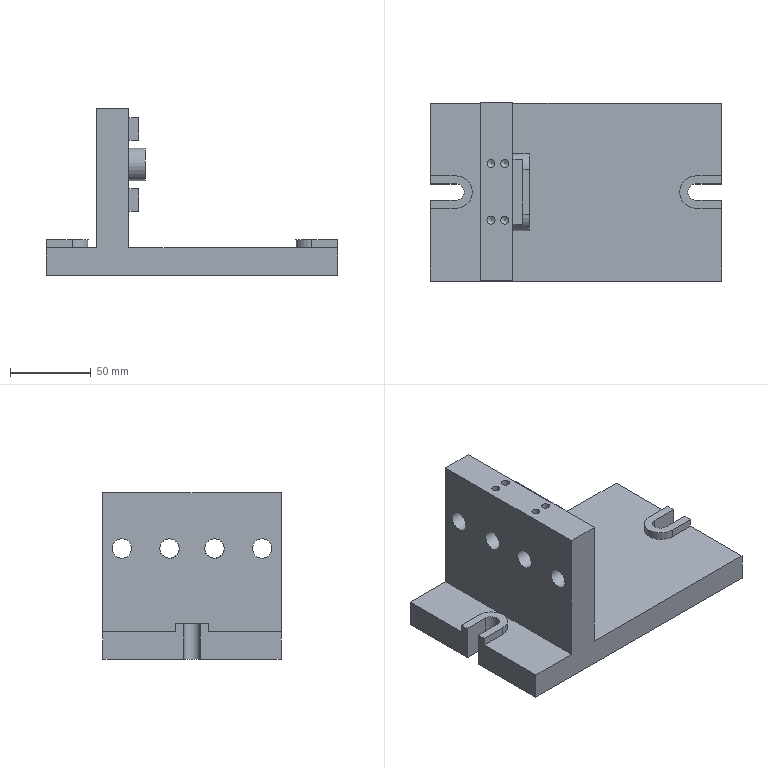Component | NX | FIXTURE_BODY | 1 solid | 61 faces | volume 524548 mm3 | plane 35 | cylinder 18 | cone 8 | commonest cylinder face diameters 4.826 x6 20 x4 12 x4 10 x2 5 x2